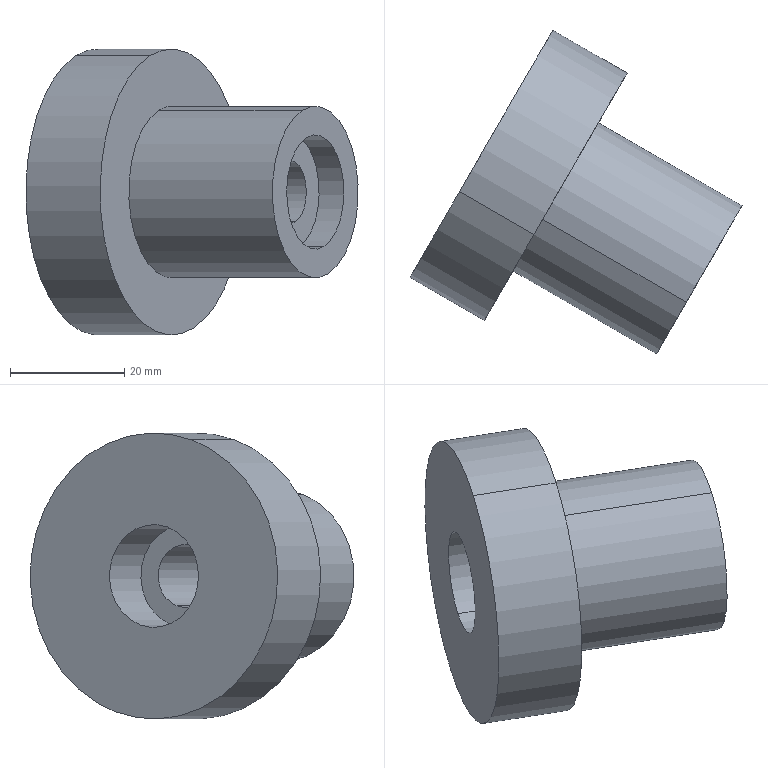Component | SolidWorks | KLHFH019EjectorPlate-1 | 1 solid | 15 faces | box 58.11 x 56.64 x 50 mm | volume 42920 mm3 | cylinder 10 | plane 5 | commonest cylinder face diameters 20 x2 18 x2 30 x2 50 x2 11 x2 | material 6061 Alloy
build123d program:
from build123d import *

# Parameters (mm, degrees)
SKETCH1_R                                          = 25
BOSS_EXTRUDE1_DEPTH                                = 15
SKETCH5_R                                          = 15
BOSS_EXTRUDE2_DEPTH                                = 29
HOLE_SIZE_ACCORDING_TO_TYPE_1_OF_HEXAG_D           = 11
HOLE_SIZE_ACCORDING_TO_TYPE_1_OF_HEXAG_CBORE_D     = 18
HOLE_SIZE_ACCORDING_TO_TYPE_1_OF_HEXAG_CBORE_DEPTH = 11
SKETCH8_R                                          = 10
CUT_EXTRUDE1_DEPTH                                 = 5


with BuildPart() as part:
    # Sketch1 → Boss-Extrude1 (new body)
    with BuildSketch(Plane.XY):
        Circle(SKETCH1_R)
    extrude(amount=BOSS_EXTRUDE1_DEPTH)

    # Sketch5 → Boss-Extrude2 (add)
    with BuildSketch(Plane(origin=(0, 0, 0), x_dir=(-1, 0, 0), z_dir=(0, 0, -1))):
        with Locations(Location((0, 0, 0), (0, 0, 180))):
            Circle(SKETCH5_R)
    extrude(amount=BOSS_EXTRUDE2_DEPTH)

    # Hole Size _according to_ Type 1 of Hexag (through all)
    with Locations(Plane.XY.offset(15)):
        with Locations((0, 0)):
            CounterBoreHole(HOLE_SIZE_ACCORDING_TO_TYPE_1_OF_HEXAG_D / 2, HOLE_SIZE_ACCORDING_TO_TYPE_1_OF_HEXAG_CBORE_D / 2, HOLE_SIZE_ACCORDING_TO_TYPE_1_OF_HEXAG_CBORE_DEPTH)

    # Sketch8 → Cut-Extrude1 (cut)
    with BuildSketch(Plane(origin=(0, 0, -29), x_dir=(-1, 0, 0), z_dir=(0, 0, -1))):
        Circle(SKETCH8_R)
    extrude(amount=-CUT_EXTRUDE1_DEPTH, mode=Mode.SUBTRACT)


solid = part.part

# Placed as in the assembly
solid = solid.moved(Location((137.649, 132.416, -405.5), (-90, -60, 175.561)))
STEP:
#1=COLOUR_RGB('',0.7922,0.8196,0.9333);
#2=FILL_AREA_STYLE_COLOUR('',#1);
#3=FILL_AREA_STYLE('',(#2));
#4=SURFACE_STYLE_FILL_AREA(#3);
#5=SURFACE_SIDE_STYLE('',(#4));
#6=SURFACE_STYLE_USAGE(.BOTH.,#5);
#7=PRESENTATION_STYLE_ASSIGNMENT((#6));
#8=CARTESIAN_POINT('',(6.178,4.637,-15.59));
#9=VERTEX_POINT('',#8);
#10=CARTESIAN_POINT('',(6.298,4.845,-16.34));
#11=VERTEX_POINT('',#10);
#12=CARTESIAN_POINT('',(6.238,4.741,-15.965));
#13=DIRECTION('',(0.866,-0.5,-0.));
#14=DIRECTION('',(0.1525,0.2642,-0.9523));
#15=AXIS2_PLACEMENT_3D('',#12,#13,#14);
#16=CIRCLE('',#15,0.3937);
#17=EDGE_CURVE('',#9,#11,#16,.T.);
#18=ORIENTED_EDGE('',*,*,#17,.F.);
#19=CARTESIAN_POINT('',(6.348,4.538,-15.59));
#20=VERTEX_POINT('',#19);
#21=CARTESIAN_POINT('',(6.178,4.637,-15.59));
#22=DIRECTION('',(0.866,-0.5,-0.));
#23=VECTOR('',#22,39.37);
#24=LINE('',#21,#23);
#25=EDGE_CURVE('',#9,#20,#24,.T.);
#26=ORIENTED_EDGE('',*,*,#25,.T.);
#27=CARTESIAN_POINT('',(6.468,4.746,-16.34));
#28=VERTEX_POINT('',#27);
#29=CARTESIAN_POINT('',(6.408,4.642,-15.965));
#30=DIRECTION('',(0.866,-0.5,-0.));
#31=DIRECTION('',(0.1525,0.2642,-0.9523));
#32=AXIS2_PLACEMENT_3D('',#29,#30,#31);
#33=CIRCLE('',#32,0.3937);
#34=EDGE_CURVE('',#20,#28,#33,.T.);
#35=ORIENTED_EDGE('',*,*,#34,.T.);
#36=CARTESIAN_POINT('',(6.298,4.845,-16.34));
#37=DIRECTION('',(0.866,-0.5,-0.));
#38=VECTOR('',#37,39.37);
#39=LINE('',#36,#38);
#40=EDGE_CURVE('',#11,#28,#39,.T.);
#41=ORIENTED_EDGE('',*,*,#40,.F.);
#42=EDGE_LOOP('',(#18,#26,#35,#41));
#43=FACE_OUTER_BOUND('',#42,.T.);
#44=CARTESIAN_POINT('',(6.238,4.741,-15.965));
#45=DIRECTION('',(0.866,-0.5,-0.));
#46=DIRECTION('',(0.1525,0.2642,-0.9523));
#47=AXIS2_PLACEMENT_3D('',#44,#45,#46);
#48=CYLINDRICAL_SURFACE('',#47,0.3937);
#49=ADVANCED_FACE('',(#43),#48,.F.);
#50=CARTESIAN_POINT('',(5.337,5.386,-16.302));
#51=VERTEX_POINT('',#50);
#52=CARTESIAN_POINT('',(5.229,5.198,-15.627));
#53=VERTEX_POINT('',#52);
#54=CARTESIAN_POINT('',(5.283,5.292,-15.965));
#55=DIRECTION('',(-0.866,0.5,0.));
#56=DIRECTION('',(-0.1525,-0.2642,0.9523));
#57=AXIS2_PLACEMENT_3D('',#54,#55,#56);
#58=CIRCLE('',#57,0.3543);
#59=EDGE_CURVE('',#51,#53,#58,.T.);
#60=ORIENTED_EDGE('',*,*,#59,.F.);
#61=CARTESIAN_POINT('',(4.962,5.602,-16.302));
#62=VERTEX_POINT('',#61);
#63=CARTESIAN_POINT('',(4.962,5.602,-16.302));
#64=DIRECTION('',(-0.866,0.5,0.));
#65=VECTOR('',#64,39.37);
#66=LINE('',#63,#65);
#67=EDGE_CURVE('',#51,#62,#66,.T.);
#68=ORIENTED_EDGE('',*,*,#67,.T.);
#69=CARTESIAN_POINT('',(4.854,5.415,-15.627));
#70=VERTEX_POINT('',#69);
#71=CARTESIAN_POINT('',(4.908,5.508,-15.965));
#72=DIRECTION('',(-0.866,0.5,0.));
#73=DIRECTION('',(-0.1525,-0.2642,0.9523));
#74=AXIS2_PLACEMENT_3D('',#71,#72,#73);
#75=CIRCLE('',#74,0.3543);
#76=EDGE_CURVE('',#62,#70,#75,.T.);
#77=ORIENTED_EDGE('',*,*,#76,.T.);
#78=CARTESIAN_POINT('',(4.854,5.415,-15.627));
#79=DIRECTION('',(-0.866,0.5,0.));
#80=VECTOR('',#79,39.37);
#81=LINE('',#78,#80);
#82=EDGE_CURVE('',#53,#70,#81,.T.);
#83=ORIENTED_EDGE('',*,*,#82,.F.);
#84=EDGE_LOOP('',(#60,#68,#77,#83));
#85=FACE_OUTER_BOUND('',#84,.T.);
#86=CARTESIAN_POINT('',(4.908,5.508,-15.965));
#87=DIRECTION('',(-0.866,0.5,0.));
#88=DIRECTION('',(-0.1525,-0.2642,0.9523));
#89=AXIS2_PLACEMENT_3D('',#86,#87,#88);
#90=CYLINDRICAL_SURFACE('',#89,0.3543);
#91=ADVANCED_FACE('',(#85),#90,.F.);
#92=CARTESIAN_POINT('',(6.498,4.798,-16.527));
#93=VERTEX_POINT('',#92);
#94=CARTESIAN_POINT('',(6.318,4.486,-15.402));
#95=VERTEX_POINT('',#94);
#96=CARTESIAN_POINT('',(6.408,4.642,-15.965));
#97=DIRECTION('',(0.866,-0.5,-0.));
#98=DIRECTION('',(0.1525,0.2642,-0.9523));
#99=AXIS2_PLACEMENT_3D('',#96,#97,#98);
#100=CIRCLE('',#99,0.5906);
#101=EDGE_CURVE('',#93,#95,#100,.T.);
#102=ORIENTED_EDGE('',*,*,#101,.F.);
#103=CARTESIAN_POINT('',(5.509,5.369,-16.527));
#104=VERTEX_POINT('',#103);
#105=CARTESIAN_POINT('',(6.498,4.798,-16.527));
#106=DIRECTION('',(-0.866,0.5,0.));
#107=VECTOR('',#106,39.37);
#108=LINE('',#105,#107);
#109=EDGE_CURVE('',#93,#104,#108,.T.);
#110=ORIENTED_EDGE('',*,*,#109,.T.);
#111=CARTESIAN_POINT('',(5.329,5.057,-15.402));
#112=VERTEX_POINT('',#111);
#113=CARTESIAN_POINT('',(5.419,5.213,-15.965));
#114=DIRECTION('',(0.866,-0.5,-0.));
#115=DIRECTION('',(-0.1525,-0.2642,0.9523));
#116=AXIS2_PLACEMENT_3D('',#113,#114,#115);
#117=CIRCLE('',#116,0.5906);
#118=EDGE_CURVE('',#104,#112,#117,.T.);
#119=ORIENTED_EDGE('',*,*,#118,.T.);
#120=CARTESIAN_POINT('',(6.318,4.486,-15.402));
#121=DIRECTION('',(-0.866,0.5,0.));
#122=VECTOR('',#121,39.37);
#123=LINE('',#120,#122);
#124=EDGE_CURVE('',#95,#112,#123,.T.);
#125=ORIENTED_EDGE('',*,*,#124,.F.);
#126=EDGE_LOOP('',(#102,#110,#119,#125));
#127=FACE_OUTER_BOUND('',#126,.T.);
#128=CARTESIAN_POINT('',(6.408,4.642,-15.965));
#129=DIRECTION('',(-0.866,0.5,0.));
#130=DIRECTION('',(-0.1525,-0.2642,0.9523));
#131=AXIS2_PLACEMENT_3D('',#128,#129,#130);
#132=CYLINDRICAL_SURFACE('',#131,0.5906);
#133=ADVANCED_FACE('',(#127),#132,.T.);
#134=CARTESIAN_POINT('',(4.758,5.248,-15.027));
#135=VERTEX_POINT('',#134);
#136=CARTESIAN_POINT('',(5.058,5.769,-16.902));
#137=VERTEX_POINT('',#136);
#138=CARTESIAN_POINT('',(4.908,5.508,-15.965));
#139=DIRECTION('',(-0.866,0.5,0.));
#140=DIRECTION('',(-0.1525,-0.2642,0.9523));
#141=AXIS2_PLACEMENT_3D('',#138,#139,#140);
#142=CIRCLE('',#141,0.9843);
#143=EDGE_CURVE('',#135,#137,#142,.T.);
#144=ORIENTED_EDGE('',*,*,#143,.F.);
#145=CARTESIAN_POINT('',(5.269,4.953,-15.027));
#146=VERTEX_POINT('',#145);
#147=CARTESIAN_POINT('',(4.758,5.248,-15.027));
#148=DIRECTION('',(0.866,-0.5,-0.));
#149=VECTOR('',#148,39.37);
#150=LINE('',#147,#149);
#151=EDGE_CURVE('',#135,#146,#150,.T.);
#152=ORIENTED_EDGE('',*,*,#151,.T.);
#153=CARTESIAN_POINT('',(5.569,5.473,-16.902));
#154=VERTEX_POINT('',#153);
#155=CARTESIAN_POINT('',(5.419,5.213,-15.965));
#156=DIRECTION('',(-0.866,0.5,0.));
#157=DIRECTION('',(-0.1525,-0.2642,0.9523));
#158=AXIS2_PLACEMENT_3D('',#155,#156,#157);
#159=CIRCLE('',#158,0.9843);
#160=EDGE_CURVE('',#146,#154,#159,.T.);
#161=ORIENTED_EDGE('',*,*,#160,.T.);
#162=CARTESIAN_POINT('',(5.058,5.769,-16.902));
#163=DIRECTION('',(0.866,-0.5,-0.));
#164=VECTOR('',#163,39.37);
#165=LINE('',#162,#164);
#166=EDGE_CURVE('',#137,#154,#165,.T.);
#167=ORIENTED_EDGE('',*,*,#166,.F.);
#168=EDGE_LOOP('',(#144,#152,#161,#167));
#169=FACE_OUTER_BOUND('',#168,.T.);
#170=CARTESIAN_POINT('',(4.908,5.508,-15.965));
#171=DIRECTION('',(0.866,-0.5,-0.));
#172=DIRECTION('',(0.1525,0.2642,-0.9523));
#173=AXIS2_PLACEMENT_3D('',#170,#171,#172);
#174=CYLINDRICAL_SURFACE('',#173,0.9843);
#175=ADVANCED_FACE('',(#169),#174,.T.);
#176=CARTESIAN_POINT('',(6.271,4.798,-16.171));
#177=VERTEX_POINT('',#176);
#178=CARTESIAN_POINT('',(6.205,4.684,-15.758));
#179=VERTEX_POINT('',#178);
#180=CARTESIAN_POINT('',(6.238,4.741,-15.965));
#181=DIRECTION('',(-0.866,0.5,0.));
#182=DIRECTION('',(0.1525,0.2642,-0.9523));
#183=AXIS2_PLACEMENT_3D('',#180,#181,#182);
#184=CIRCLE('',#183,0.2165);
#185=EDGE_CURVE('',#177,#179,#184,.T.);
#186=ORIENTED_EDGE('',*,*,#185,.F.);
#187=CARTESIAN_POINT('',(5.316,5.349,-16.171));
#188=VERTEX_POINT('',#187);
#189=CARTESIAN_POINT('',(4.941,5.566,-16.171));
#190=DIRECTION('',(-0.866,0.5,0.));
#191=VECTOR('',#190,39.37);
#192=LINE('',#189,#191);
#193=EDGE_CURVE('',#177,#188,#192,.T.);
#194=ORIENTED_EDGE('',*,*,#193,.T.);
#195=CARTESIAN_POINT('',(5.25,5.235,-15.758));
#196=VERTEX_POINT('',#195);
#197=CARTESIAN_POINT('',(5.283,5.292,-15.965));
#198=DIRECTION('',(-0.866,0.5,0.));
#199=DIRECTION('',(-0.1525,-0.2642,0.9523));
#200=AXIS2_PLACEMENT_3D('',#197,#198,#199);
#201=CIRCLE('',#200,0.2165);
#202=EDGE_CURVE('',#188,#196,#201,.T.);
#203=ORIENTED_EDGE('',*,*,#202,.T.);
#204=CARTESIAN_POINT('',(4.875,5.451,-15.758));
#205=DIRECTION('',(-0.866,0.5,0.));
#206=VECTOR('',#205,39.37);
#207=LINE('',#204,#206);
#208=EDGE_CURVE('',#179,#196,#207,.T.);
#209=ORIENTED_EDGE('',*,*,#208,.F.);
#210=EDGE_LOOP('',(#186,#194,#203,#209));
#211=FACE_OUTER_BOUND('',#210,.T.);
#212=CARTESIAN_POINT('',(4.908,5.508,-15.965));
#213=DIRECTION('',(-0.866,0.5,0.));
#214=DIRECTION('',(-0.1525,-0.2642,0.9523));
#215=AXIS2_PLACEMENT_3D('',#212,#213,#214);
#216=CYLINDRICAL_SURFACE('',#215,0.2165);
#217=ADVANCED_FACE('',(#211),#216,.F.);
#218=ORIENTED_EDGE('',*,*,#193,.F.);
#219=CARTESIAN_POINT('',(6.238,4.741,-15.965));
#220=DIRECTION('',(-0.866,0.5,0.));
#221=DIRECTION('',(0.1525,0.2642,-0.9523));
#222=AXIS2_PLACEMENT_3D('',#219,#220,#221);
#223=CIRCLE('',#222,0.2165);
#224=EDGE_CURVE('',#179,#177,#223,.T.);
#225=ORIENTED_EDGE('',*,*,#224,.F.);
#226=ORIENTED_EDGE('',*,*,#208,.T.);
#227=CARTESIAN_POINT('',(5.283,5.292,-15.965));
#228=DIRECTION('',(-0.866,0.5,0.));
#229=DIRECTION('',(-0.1525,-0.2642,0.9523));
#230=AXIS2_PLACEMENT_3D('',#227,#228,#229);
#231=CIRCLE('',#230,0.2165);
#232=EDGE_CURVE('',#196,#188,#231,.T.);
#233=ORIENTED_EDGE('',*,*,#232,.T.);
#234=EDGE_LOOP('',(#218,#225,#226,#233));
#235=FACE_OUTER_BOUND('',#234,.T.);
#236=CARTESIAN_POINT('',(4.908,5.508,-15.965));
#237=DIRECTION('',(-0.866,0.5,0.));
#238=DIRECTION('',(-0.1525,-0.2642,0.9523));
#239=AXIS2_PLACEMENT_3D('',#236,#237,#238);
#240=CYLINDRICAL_SURFACE('',#239,0.2165);
#241=ADVANCED_FACE('',(#235),#240,.F.);
#242=CARTESIAN_POINT('',(5.419,5.213,-15.965));
#243=DIRECTION('',(-0.866,0.5,0.));
#244=DIRECTION('',(-0.1525,-0.2642,0.9523));
#245=AXIS2_PLACEMENT_3D('',#242,#243,#244);
#246=CIRCLE('',#245,0.9843);
#247=EDGE_CURVE('',#154,#146,#246,.T.);
#248=ORIENTED_EDGE('',*,*,#247,.F.);
#249=ORIENTED_EDGE('',*,*,#160,.F.);
#250=EDGE_LOOP('',(#248,#249));
#251=FACE_OUTER_BOUND('',#250,.T.);
#252=CARTESIAN_POINT('',(5.419,5.213,-15.965));
#253=DIRECTION('',(0.866,-0.5,-0.));
#254=DIRECTION('',(-0.1525,-0.2642,0.9523));
#255=AXIS2_PLACEMENT_3D('',#252,#253,#254);
#256=CIRCLE('',#255,0.5906);
#257=EDGE_CURVE('',#112,#104,#256,.T.);
#258=ORIENTED_EDGE('',*,*,#257,.F.);
#259=ORIENTED_EDGE('',*,*,#118,.F.);
#260=EDGE_LOOP('',(#258,#259));
#261=FACE_BOUND('',#260,.T.);
#262=CARTESIAN_POINT('',(5.419,5.213,-15.965));
#263=DIRECTION('',(-0.866,0.5,0.));
#264=DIRECTION('',(-0.1525,-0.2642,0.9523));
#265=AXIS2_PLACEMENT_3D('',#262,#263,#264);
#266=PLANE('',#265);
#267=ADVANCED_FACE('',(#251,#261),#266,.F.);
#268=ORIENTED_EDGE('',*,*,#151,.F.);
#269=CARTESIAN_POINT('',(4.908,5.508,-15.965));
#270=DIRECTION('',(-0.866,0.5,0.));
#271=DIRECTION('',(-0.1525,-0.2642,0.9523));
#272=AXIS2_PLACEMENT_3D('',#269,#270,#271);
#273=CIRCLE('',#272,0.9843);
#274=EDGE_CURVE('',#137,#135,#273,.T.);
#275=ORIENTED_EDGE('',*,*,#274,.F.);
#276=ORIENTED_EDGE('',*,*,#166,.T.);
#277=ORIENTED_EDGE('',*,*,#247,.T.);
#278=EDGE_LOOP('',(#268,#275,#276,#277));
#279=FACE_OUTER_BOUND('',#278,.T.);
#280=CARTESIAN_POINT('',(4.908,5.508,-15.965));
#281=DIRECTION('',(0.866,-0.5,-0.));
#282=DIRECTION('',(0.1525,0.2642,-0.9523));
#283=AXIS2_PLACEMENT_3D('',#280,#281,#282);
#284=CYLINDRICAL_SURFACE('',#283,0.9843);
#285=ADVANCED_FACE('',(#279),#284,.T.);
#286=CARTESIAN_POINT('',(4.908,5.508,-15.965));
#287=DIRECTION('',(-0.866,0.5,0.));
#288=DIRECTION('',(-0.1525,-0.2642,0.9523));
#289=AXIS2_PLACEMENT_3D('',#286,#287,#288);
#290=CIRCLE('',#289,0.3543);
#291=EDGE_CURVE('',#70,#62,#290,.T.);
#292=ORIENTED_EDGE('',*,*,#291,.F.);
#293=ORIENTED_EDGE('',*,*,#76,.F.);
#294=EDGE_LOOP('',(#292,#293));
#295=FACE_BOUND('',#294,.T.);
#296=ORIENTED_EDGE('',*,*,#274,.T.);
#297=ORIENTED_EDGE('',*,*,#143,.T.);
#298=EDGE_LOOP('',(#296,#297));
#299=FACE_OUTER_BOUND('',#298,.T.);
#300=CARTESIAN_POINT('',(4.908,5.508,-15.965));
#301=DIRECTION('',(-0.866,0.5,0.));
#302=DIRECTION('',(-0.1525,-0.2642,0.9523));
#303=AXIS2_PLACEMENT_3D('',#300,#301,#302);
#304=PLANE('',#303);
#305=ADVANCED_FACE('',(#295,#299),#304,.T.);
#306=ORIENTED_EDGE('',*,*,#109,.F.);
#307=CARTESIAN_POINT('',(6.408,4.642,-15.965));
#308=DIRECTION('',(0.866,-0.5,-0.));
#309=DIRECTION('',(0.1525,0.2642,-0.9523));
#310=AXIS2_PLACEMENT_3D('',#307,#308,#309);
#311=CIRCLE('',#310,0.5906);
#312=EDGE_CURVE('',#95,#93,#311,.T.);
#313=ORIENTED_EDGE('',*,*,#312,.F.);
#314=ORIENTED_EDGE('',*,*,#124,.T.);
#315=ORIENTED_EDGE('',*,*,#257,.T.);
#316=EDGE_LOOP('',(#306,#313,#314,#315));
#317=FACE_OUTER_BOUND('',#316,.T.);
#318=CARTESIAN_POINT('',(6.408,4.642,-15.965));
#319=DIRECTION('',(-0.866,0.5,0.));
#320=DIRECTION('',(-0.1525,-0.2642,0.9523));
#321=AXIS2_PLACEMENT_3D('',#318,#319,#320);
#322=CYLINDRICAL_SURFACE('',#321,0.5906);
#323=ADVANCED_FACE('',(#317),#322,.T.);
#324=CARTESIAN_POINT('',(6.408,4.642,-15.965));
#325=DIRECTION('',(0.866,-0.5,-0.));
#326=DIRECTION('',(0.1525,0.2642,-0.9523));
#327=AXIS2_PLACEMENT_3D('',#324,#325,#326);
#328=CIRCLE('',#327,0.3937);
#329=EDGE_CURVE('',#28,#20,#328,.T.);
#330=ORIENTED_EDGE('',*,*,#329,.F.);
#331=ORIENTED_EDGE('',*,*,#34,.F.);
#332=EDGE_LOOP('',(#330,#331));
#333=FACE_BOUND('',#332,.T.);
#334=ORIENTED_EDGE('',*,*,#312,.T.);
#335=ORIENTED_EDGE('',*,*,#101,.T.);
#336=EDGE_LOOP('',(#334,#335));
#337=FACE_OUTER_BOUND('',#336,.T.);
#338=CARTESIAN_POINT('',(6.408,4.642,-15.965));
#339=DIRECTION('',(0.866,-0.5,-0.));
#340=DIRECTION('',(0.1525,0.2642,-0.9523));
#341=AXIS2_PLACEMENT_3D('',#338,#339,#340);
#342=PLANE('',#341);
#343=ADVANCED_FACE('',(#333,#337),#342,.T.);
#344=ORIENTED_EDGE('',*,*,#232,.F.);
#345=ORIENTED_EDGE('',*,*,#202,.F.);
#346=EDGE_LOOP('',(#344,#345));
#347=FACE_BOUND('',#346,.T.);
#348=CARTESIAN_POINT('',(5.283,5.292,-15.965));
#349=DIRECTION('',(-0.866,0.5,0.));
#350=DIRECTION('',(-0.1525,-0.2642,0.9523));
#351=AXIS2_PLACEMENT_3D('',#348,#349,#350);
#352=CIRCLE('',#351,0.3543);
#353=EDGE_CURVE('',#53,#51,#352,.T.);
#354=ORIENTED_EDGE('',*,*,#353,.T.);
#355=ORIENTED_EDGE('',*,*,#59,.T.);
#356=EDGE_LOOP('',(#354,#355));
#357=FACE_OUTER_BOUND('',#356,.T.);
#358=CARTESIAN_POINT('',(5.25,5.235,-15.758));
#359=DIRECTION('',(0.866,-0.5,-0.));
#360=DIRECTION('',(0.1525,0.2642,-0.9523));
#361=AXIS2_PLACEMENT_3D('',#358,#359,#360);
#362=PLANE('',#361);
#363=ADVANCED_FACE('',(#347,#357),#362,.F.);
#364=ORIENTED_EDGE('',*,*,#67,.F.);
#365=ORIENTED_EDGE('',*,*,#353,.F.);
#366=ORIENTED_EDGE('',*,*,#82,.T.);
#367=ORIENTED_EDGE('',*,*,#291,.T.);
#368=EDGE_LOOP('',(#364,#365,#366,#367));
#369=FACE_OUTER_BOUND('',#368,.T.);
#370=CARTESIAN_POINT('',(4.908,5.508,-15.965));
#371=DIRECTION('',(-0.866,0.5,0.));
#372=DIRECTION('',(-0.1525,-0.2642,0.9523));
#373=AXIS2_PLACEMENT_3D('',#370,#371,#372);
#374=CYLINDRICAL_SURFACE('',#373,0.3543);
#375=ADVANCED_FACE('',(#369),#374,.F.);
#376=CARTESIAN_POINT('',(6.238,4.741,-15.965));
#377=DIRECTION('',(0.866,-0.5,-0.));
#378=DIRECTION('',(0.1525,0.2642,-0.9523));
#379=AXIS2_PLACEMENT_3D('',#376,#377,#378);
#380=CIRCLE('',#379,0.3937);
#381=EDGE_CURVE('',#11,#9,#380,.T.);
#382=ORIENTED_EDGE('',*,*,#381,.T.);
#383=ORIENTED_EDGE('',*,*,#17,.T.);
#384=EDGE_LOOP('',(#382,#383));
#385=FACE_OUTER_BOUND('',#384,.T.);
#386=ORIENTED_EDGE('',*,*,#224,.T.);
#387=ORIENTED_EDGE('',*,*,#185,.T.);
#388=EDGE_LOOP('',(#386,#387));
#389=FACE_BOUND('',#388,.T.);
#390=CARTESIAN_POINT('',(6.238,4.741,-15.965));
#391=DIRECTION('',(0.866,-0.5,-0.));
#392=DIRECTION('',(0.1525,0.2642,-0.9523));
#393=AXIS2_PLACEMENT_3D('',#390,#391,#392);
#394=PLANE('',#393);
#395=ADVANCED_FACE('',(#385,#389),#394,.T.);
#396=ORIENTED_EDGE('',*,*,#25,.F.);
#397=ORIENTED_EDGE('',*,*,#381,.F.);
#398=ORIENTED_EDGE('',*,*,#40,.T.);
#399=ORIENTED_EDGE('',*,*,#329,.T.);
#400=EDGE_LOOP('',(#396,#397,#398,#399));
#401=FACE_OUTER_BOUND('',#400,.T.);
#402=CARTESIAN_POINT('',(6.238,4.741,-15.965));
#403=DIRECTION('',(0.866,-0.5,-0.));
#404=DIRECTION('',(0.1525,0.2642,-0.9523));
#405=AXIS2_PLACEMENT_3D('',#402,#403,#404);
#406=CYLINDRICAL_SURFACE('',#405,0.3937);
#407=ADVANCED_FACE('',(#401),#406,.F.);
#408=CLOSED_SHELL('',(#49,#91,#133,#175,#217,#241,#267,#285,#305,#323,#343,#363,#375,#395,#407));
#409=MANIFOLD_SOLID_BREP('',#408);
#410=STYLED_ITEM('',(#7),#409);
#411=PRESENTATION_LAYER_ASSIGNMENT('','',(#410));
#412=CARTESIAN_POINT('',(0.,0.,0.));
#413=DIRECTION('',(0.,0.,1.));
#414=DIRECTION('',(1.,0.,0.));
#415=AXIS2_PLACEMENT_3D('',#412,#413,#414);
#416=(LENGTH_UNIT()NAMED_UNIT(*)SI_UNIT($,.METRE.));
#417=LENGTH_MEASURE_WITH_UNIT(LENGTH_MEASURE(0.0254),#416);
#418=DIMENSIONAL_EXPONENTS(1.,0.,0.,0.,0.,0.,0.);
#419=(CONVERSION_BASED_UNIT('',#417)LENGTH_UNIT()NAMED_UNIT(#418));
#420=UNCERTAINTY_MEASURE_WITH_UNIT(LENGTH_MEASURE(0.00001),#419,'','');
#421=(NAMED_UNIT(*)PLANE_ANGLE_UNIT()SI_UNIT($,.RADIAN.));
#422=(NAMED_UNIT(*)SI_UNIT($,.STERADIAN.)SOLID_ANGLE_UNIT());
#423=(GEOMETRIC_REPRESENTATION_CONTEXT(3)GLOBAL_UNCERTAINTY_ASSIGNED_CONTEXT((#420))GLOBAL_UNIT_ASSIGNED_CONTEXT((#419,#421,#422))REPRESENTATION_CONTEXT('',''));
#424=ADVANCED_BREP_SHAPE_REPRESENTATION('',(#409,#415),#423);
#425=(LENGTH_UNIT()NAMED_UNIT(*)SI_UNIT($,.METRE.));
#426=LENGTH_MEASURE_WITH_UNIT(LENGTH_MEASURE(0.0254),#425);
#427=DIMENSIONAL_EXPONENTS(1.,0.,0.,0.,0.,0.,0.);
#428=(CONVERSION_BASED_UNIT('',#426)LENGTH_UNIT()NAMED_UNIT(#427));
#429=UNCERTAINTY_MEASURE_WITH_UNIT(LENGTH_MEASURE(0.00001),#428,'','');
#430=(NAMED_UNIT(*)PLANE_ANGLE_UNIT()SI_UNIT($,.RADIAN.));
#431=(NAMED_UNIT(*)SI_UNIT($,.STERADIAN.)SOLID_ANGLE_UNIT());
#432=(GEOMETRIC_REPRESENTATION_CONTEXT(3)GLOBAL_UNCERTAINTY_ASSIGNED_CONTEXT((#429))GLOBAL_UNIT_ASSIGNED_CONTEXT((#428,#430,#431))REPRESENTATION_CONTEXT('',''));
#433=MECHANICAL_DESIGN_GEOMETRIC_PRESENTATION_REPRESENTATION('',(#410),#432);